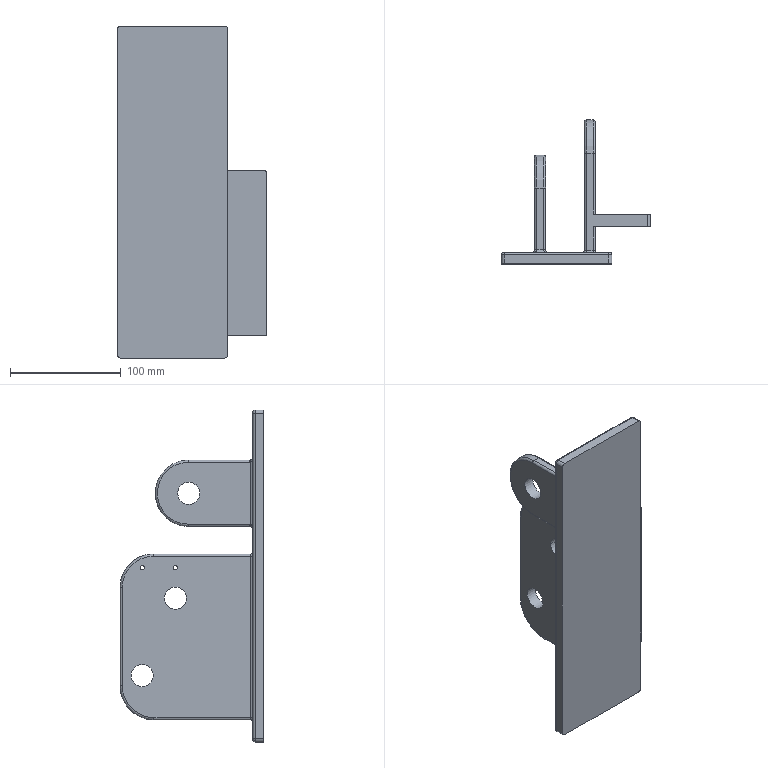Component | NX | BASE | 1 solid | 79 faces | volume 599201 mm3 | cylinder 38 | plane 19 | torus 14 | spline 8 | commonest cylinder face diameters 4 x24 6 x7 20 x4 60 x1 61.295 x1 60.162 x1